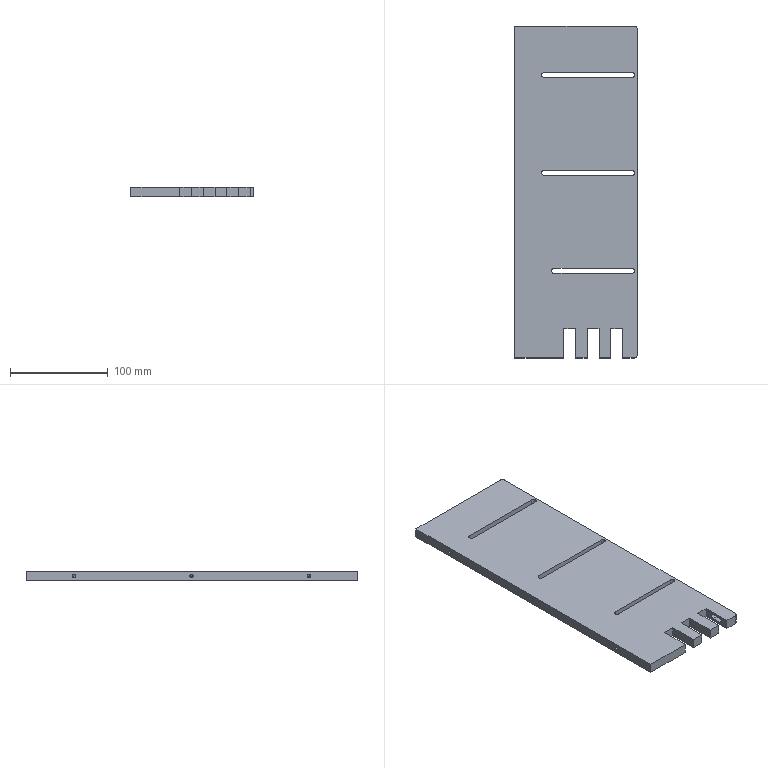Component | SolidWorks | SecondGenerationFour-sidedLabelingFeedingFrontBaffle-1 | 1 solid | 51 faces | box 125 x 339 x 10 mm | volume 397777 mm3 | plane 26 | cylinder 19 | cone 6 | commonest cylinder face diameters 5 x9 3.3 x6 5.2 x2 6 x2
build123d program:
from build123d import *

# Parameters (mm, degrees)
SKETCH1_W             = 10
SKETCH1_H             = 339
BOSS_EXTRUDE1_DEPTH   = 125
M4_TAPPED_HOLE1_D     = 3.3
M4_TAPPED_HOLE1_DEPTH = 17.1
M4_TAPPED_HOLE1_TIP   = 0.9914
SKETCH5_W             = 12
SKETCH5_H             = 55.159
SKETCH5_H_2           = 47.484
CUT_EXTRUDE1_DEPTH    = 362.45
CUT_EXTRUDE2_DEPTH    = 16
FILLET1_R             = 3
CUT_EXTRUDE3_DEPTH    = 362.45
CUT_EXTRUDE4_DEPTH    = 362.45


with BuildPart() as part:
    # Sketch1 → Boss-Extrude1 (new body)
    with BuildSketch(Plane.XY):
        with Locations((5, 169.5)):
            Rectangle(SKETCH1_W, SKETCH1_H)
    extrude(amount=BOSS_EXTRUDE1_DEPTH)

    # M4 Tapped Hole1
    with Locations(Plane(origin=(0, 0, 0), x_dir=(-1, 0, 0), z_dir=(0, 0, -1))):
        with Locations((-5, 290), (-5, 170), (-5, 50)):
            Hole(M4_TAPPED_HOLE1_D / 2, depth=M4_TAPPED_HOLE1_DEPTH)
            with Locations((0, 0, -(M4_TAPPED_HOLE1_DEPTH + M4_TAPPED_HOLE1_TIP / 2))):  # 118° drill point
                Cone(0, M4_TAPPED_HOLE1_D / 2, M4_TAPPED_HOLE1_TIP, mode=Mode.SUBTRACT)

    # Sketch5 → Cut-Extrude1 (cut, through all)
    with BuildSketch(Plane.ZY):
        with Locations((80, 2.42)):
            Rectangle(SKETCH5_W, SKETCH5_H)
        with Locations((104, 2.42)):
            Rectangle(SKETCH5_W, SKETCH5_H)
        with Locations((56, 6.258)):
            Rectangle(SKETCH5_W, SKETCH5_H_2)
    extrude(amount=-CUT_EXTRUDE1_DEPTH, mode=Mode.SUBTRACT)

    # Sketch6 → Cut-Extrude2 (cut)
    with BuildSketch(Plane.XY.offset(125)):
        with BuildLine():
            Line((2.4, 10), (2.4, 20))
            ThreePointArc((2.4, 20), (5, 22.6), (7.6, 20))
            Line((7.6, 20), (7.6, 10))
            ThreePointArc((7.6, 10), (5, 7.4), (2.4, 10))
        make_face()
    extrude(amount=-CUT_EXTRUDE2_DEPTH, mode=Mode.SUBTRACT)

    # Fillet1
    fillet1_edges = [part.edges().sort_by_distance(p)[0] for p in [
        (5, 0, 125),
        (5, 339, 125),
    ]]
    fillet(fillet1_edges, radius=FILLET1_R)

    # Sketch7 → Cut-Extrude3 (cut, through all)
    with BuildSketch(Plane(origin=(10, 0, 0), x_dir=(0, 0, -1), z_dir=(1, 0, 0))):
        with BuildLine():
            Line((-120, 291.5), (-30, 291.5))
            ThreePointArc((-30, 291.5), (-27.5, 289), (-30, 286.5))
            Line((-30, 286.5), (-120, 286.5))
            ThreePointArc((-120, 286.5), (-122.5, 289), (-120, 291.5))
        make_face()
        with BuildLine():
            Line((-120, 191.5), (-30, 191.5))
            ThreePointArc((-30, 191.5), (-27.5, 189), (-30, 186.5))
            Line((-30, 186.5), (-120, 186.5))
            ThreePointArc((-120, 186.5), (-122.5, 189), (-120, 191.5))
        make_face()
    extrude(amount=-CUT_EXTRUDE3_DEPTH, mode=Mode.SUBTRACT)

    # Sketch8 → Cut-Extrude4 (cut, through all)
    with BuildSketch(Plane(origin=(10, 0, 0), x_dir=(0, 0, -1), z_dir=(1, 0, 0))):
        with BuildLine():
            Line((-120, 91.5), (-40, 91.5))
            ThreePointArc((-40, 91.5), (-37.5, 89), (-40, 86.5))
            Line((-40, 86.5), (-120, 86.5))
            ThreePointArc((-120, 86.5), (-122.5, 89), (-120, 91.5))
        make_face()
    extrude(amount=-CUT_EXTRUDE4_DEPTH, mode=Mode.SUBTRACT)


solid = part.part

# Placed as in the assembly
solid = solid.moved(Location((-70.027, 52.863, -114), (0, 90, 0)))